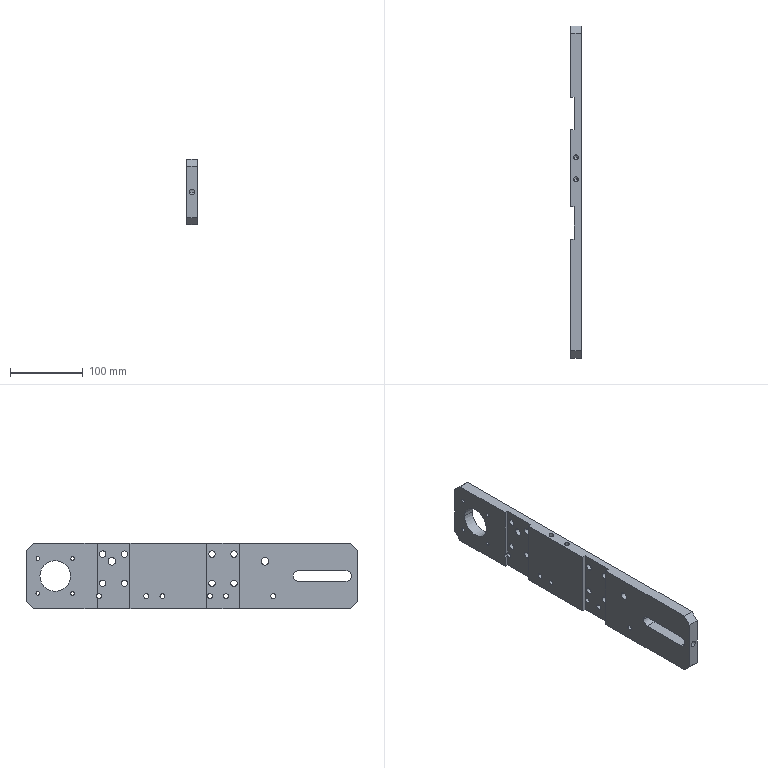Component | SolidWorks | UpperSideBeltXG-XG1-1_UpperRollerMountingPlateAXG-XG1-1 | 1 solid | 92 faces | box 15 x 455 x 90 mm | volume 516495 mm3 | cylinder 51 | plane 21 | cone 20 | commonest cylinder face diameters 6.8 x16 9 x16 5 x8 10.2 x4 15 x3 8.2 x2 42 x2
build123d program:
from build123d import *

# Parameters (mm, degrees)
SKETCH1_W                                           = 455
SKETCH1_H                                           = 90
BOSS_EXTRUDE1_DEPTH                                 = 7.5
TAPERED_COUNTERSUNK_HOLE_FOR_M8_HEXAGON_D           = 9
TAPERED_COUNTERSUNK_HOLE_FOR_M8_HEXAGON_CSINK_D     = 17.92
TAPERED_COUNTERSUNK_HOLE_FOR_M8_HEXAGON_CSINK_ANGLE = 90
M8_TAPPED_HOLE1_D                                   = 6.8
SKETCH8_R                                           = 21
CUT_EXTRUDE1_DEPTH                                  = 15
M6_TAPPED_HOLE2_D                                   = 5
CIRPATTERN1_COUNT                                   = 4
CUT_EXTRUDE2_DEPTH                                  = 15
M8_TAPPED_HOLE2_D                                   = 6.8
M8_TAPPED_HOLE2_DEPTH                               = 22.25
M8_TAPPED_HOLE2_TIP                                 = 2.043
M12_TAPPED_HOLE1_D                                  = 10.2
CHAMFER1_SIZE                                       = 10
CUT_EXTRUDE3_REACH                                  = 459.281
CUT_EXTRUDE3_END_RADIUS                             = 7.5
SKETCH21_R                                          = 4.1
SKETCH22_W                                          = 45
SKETCH22_H                                          = 19.827
SKETCH22_H_2                                        = 22.728
CUT_EXTRUDE4_DEPTH                                  = 245.77


with BuildPart() as part:
    # Sketch1 → Boss-Extrude1 (new, symmetric)
    with BuildSketch(Plane.XY):
        Rectangle(SKETCH1_W, SKETCH1_H)
    extrude(amount=BOSS_EXTRUDE1_DEPTH, both=True)

    # Tapered Countersunk Hole for M8 Hexagon (through all)
    with Locations(Plane.XY.offset(7.5)):
        with Locations((92.5, 30), (92.5, -10), (122.5, 30), (122.5, -10), (-27.5, -10), (-27.5, 30), (-57.5, 30), (-57.5, -10)):
            CounterSinkHole(TAPERED_COUNTERSUNK_HOLE_FOR_M8_HEXAGON_D / 2, TAPERED_COUNTERSUNK_HOLE_FOR_M8_HEXAGON_CSINK_D / 2, counter_sink_angle=TAPERED_COUNTERSUNK_HOLE_FOR_M8_HEXAGON_CSINK_ANGLE)

    # M8 Tapped Hole1 (through all)
    with Locations(Plane.XY.offset(7.5)):
        with Locations((62.5, -27.5), (40.5, -27.5), (-24.5, -27.5), (-46.5, -27.5), (127.5, -27.5), (-111.5, -27.5)):
            Hole(M8_TAPPED_HOLE1_D / 2)

    # Sketch8 → Cut-Extrude1 (cut)
    with BuildSketch(Plane.XY.offset(7.5)):
        with Locations((187.5, 0)):
            Circle(SKETCH8_R)
    extrude(amount=-CUT_EXTRUDE1_DEPTH, mode=Mode.SUBTRACT)

    # M6 Tapped Hole2 (through all)
    with Locations(Plane.XY.offset(7.5)):
        with Locations((163.635, 23.865)):
            m6_tapped_hole2 = Hole(M6_TAPPED_HOLE2_D / 2)

    # CirPattern1: M6 Tapped Hole2 ×4 about axis
    cirpattern1_axis = Axis((187.5, 0, 0), (0, 0, 1))
    for i in range(1, CIRPATTERN1_COUNT):
        add(m6_tapped_hole2.rotate(cirpattern1_axis, i * 360 / CIRPATTERN1_COUNT), mode=Mode.SUBTRACT)

    # Sketch11 → Cut-Extrude2 (cut)
    with BuildSketch(Plane.XY.offset(7.5)):
        with BuildLine():
            Line((-211, 7.5), (-146, 7.5))
            ThreePointArc((-146, 7.5), (-138.5, 0), (-146, -7.5))
            Line((-146, -7.5), (-211, -7.5))
            ThreePointArc((-211, -7.5), (-218.5, 0), (-211, 7.5))
        make_face()
    extrude(amount=-CUT_EXTRUDE2_DEPTH, mode=Mode.SUBTRACT)

    # M8 Tapped Hole2
    with Locations(Plane(origin=(0, 45, 0), x_dir=(1, 0, 0), z_dir=(0, 1, 0))):
        with Locations((47.5, 0), (17.5, 0)):
            Hole(M8_TAPPED_HOLE2_D / 2, depth=M8_TAPPED_HOLE2_DEPTH)
            with Locations((0, 0, -(M8_TAPPED_HOLE2_DEPTH + M8_TAPPED_HOLE2_TIP / 2))):  # 118° drill point
                Cone(0, M8_TAPPED_HOLE2_D / 2, M8_TAPPED_HOLE2_TIP, mode=Mode.SUBTRACT)

    # M12 Tapped Hole1 (through all)
    with Locations(Plane(origin=(0, 0, -7.5), x_dir=(1, 0, 0), z_dir=(0, 0, -1))):
        with Locations((-100, -20), (110, -20)):
            Hole(M12_TAPPED_HOLE1_D / 2)

    # Chamfer1
    chamfer1_edges = [part.edges().sort_by_distance(p)[0] for p in [
        (-227.5, 45, 0),
        (227.5, 45, 0),
        (227.5, -45, 0),
        (-227.5, -45, 0),
    ]]
    chamfer(chamfer1_edges, length=CHAMFER1_SIZE)

    # Cut-Extrude3: up to this cylinder (the profile starts outside it)
    cut_extrude3_end = Plane(origin=(-211, 0, 0), z_dir=(0, 0, 1)) * Cylinder(CUT_EXTRUDE3_END_RADIUS, 934.562, mode=Mode.PRIVATE)
    # Sketch21 → Cut-Extrude3 (cut, up to the surface)
    with BuildSketch(Plane.ZY.offset(227.5), mode=Mode.PRIVATE) as cut_extrude3_sk1:
        Circle(SKETCH21_R)
    cut_extrude3_tool1 = extrude(cut_extrude3_sk1.sketch, amount=-CUT_EXTRUDE3_REACH, mode=Mode.PRIVATE) - cut_extrude3_end
    add(cut_extrude3_tool1.solids().sort_by_distance((-227.5, 0, 0))[0], mode=Mode.SUBTRACT)

    # Sketch22 → Cut-Extrude4 (cut, through all)
    with BuildSketch(Plane(origin=(0, 45, 0), x_dir=(1, 0, 0), z_dir=(0, 1, 0))):
        with Locations((-42.5, 12.414)):
            Rectangle(SKETCH22_W, SKETCH22_H)
        with Locations((107.5, 13.864)):
            Rectangle(SKETCH22_W, SKETCH22_H_2)
    extrude(amount=-CUT_EXTRUDE4_DEPTH, mode=Mode.SUBTRACT)


solid = part.part

# Placed as in the assembly
solid = solid.moved(Location((-323.72, 437.5, 263), (90, 90, 0)))